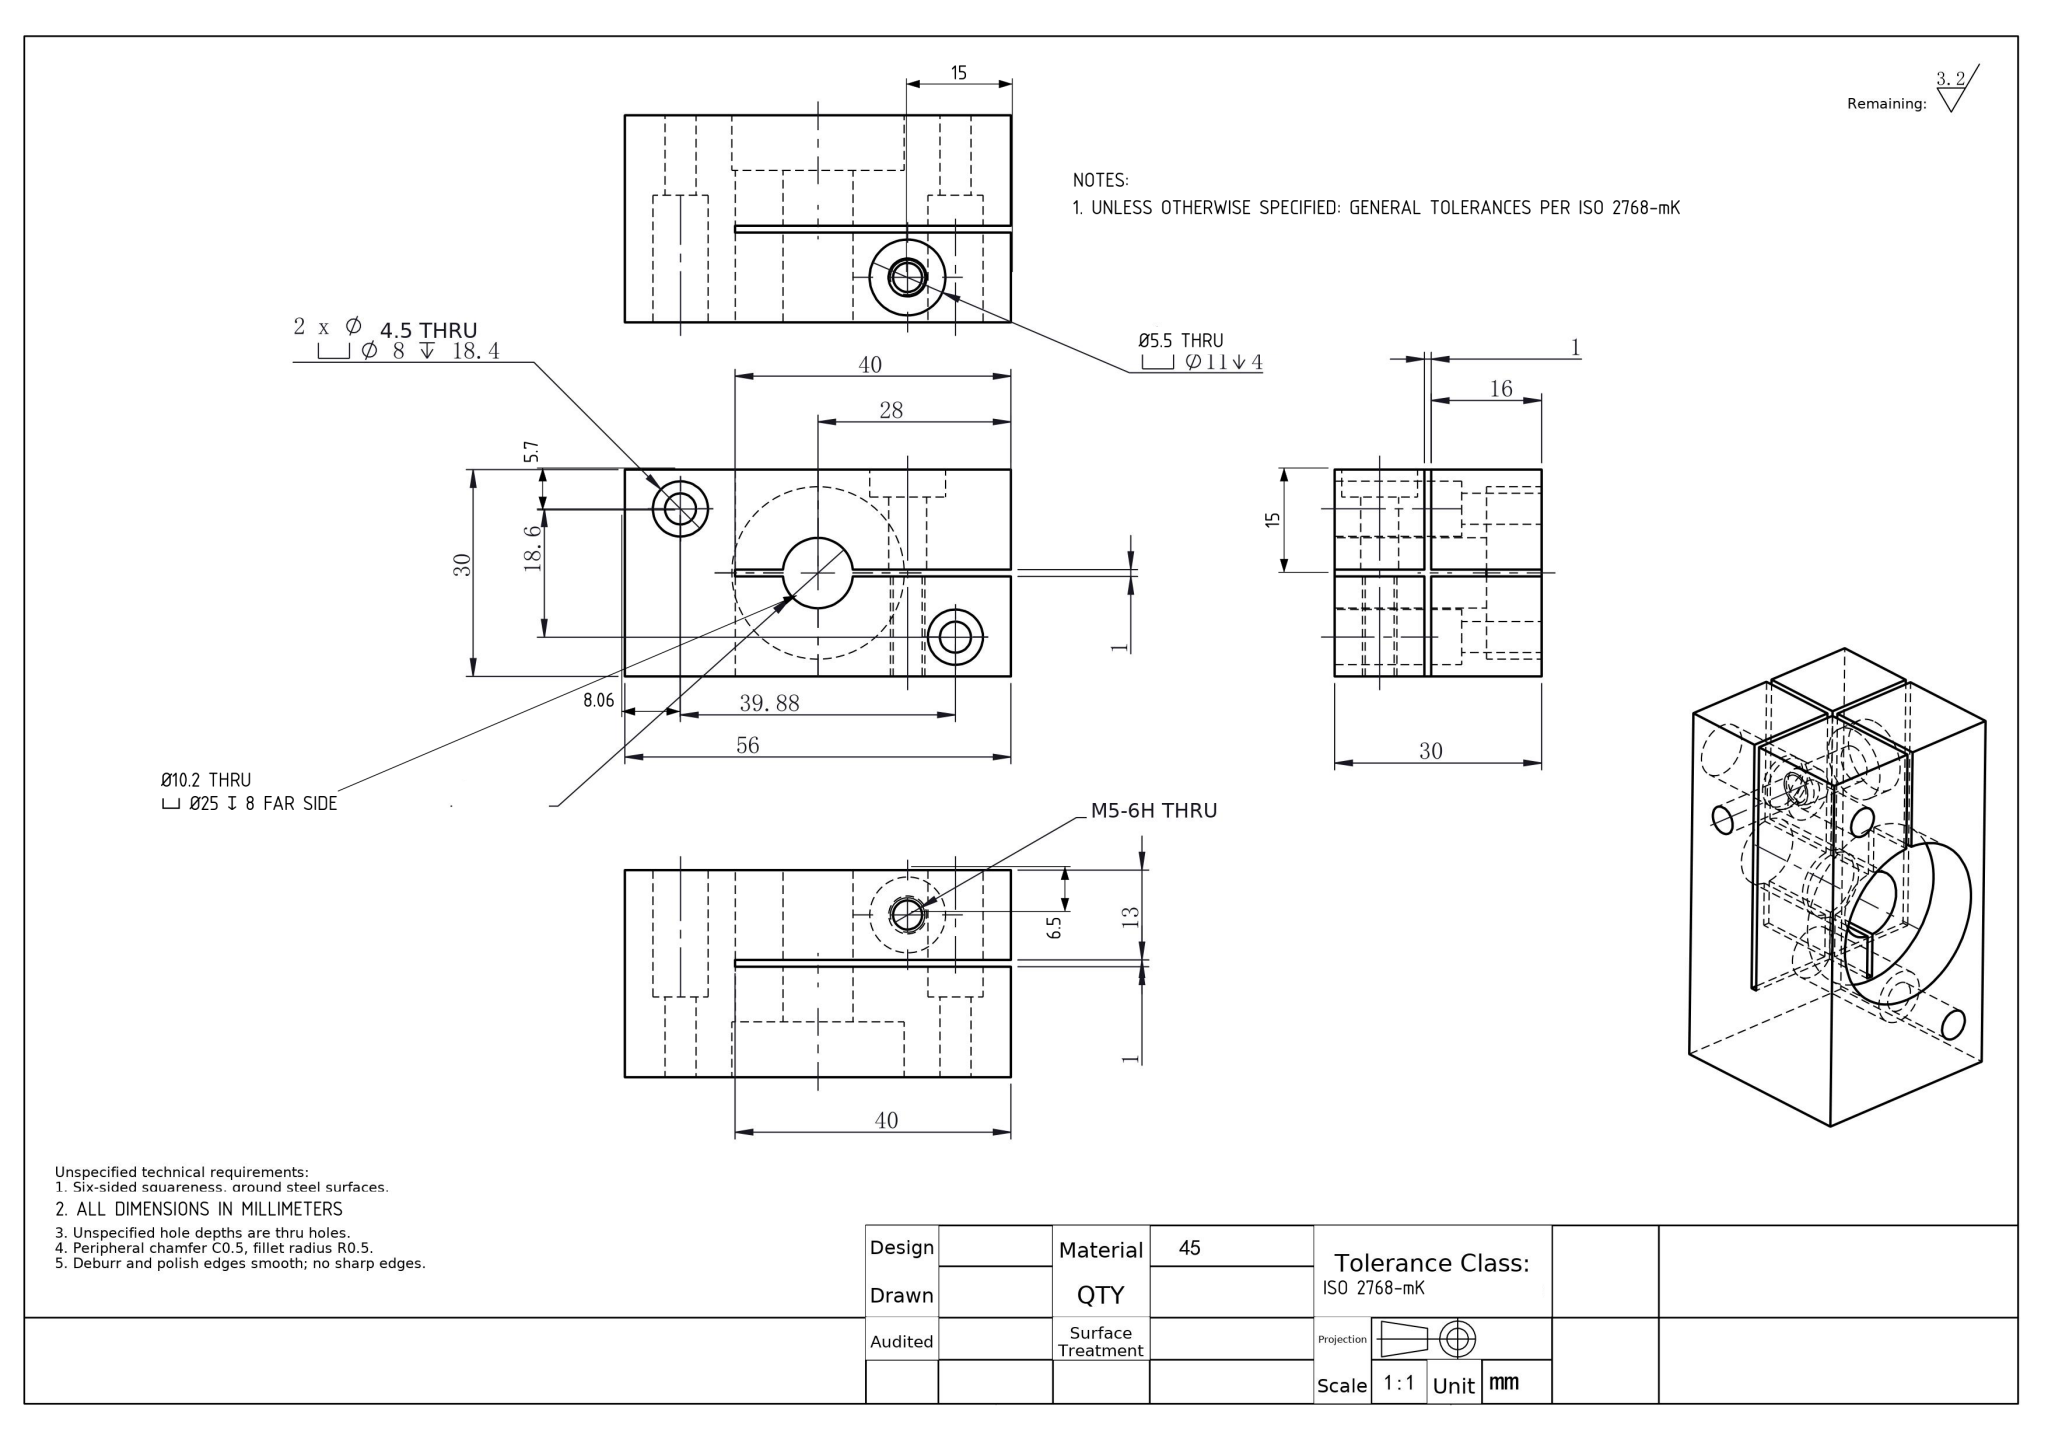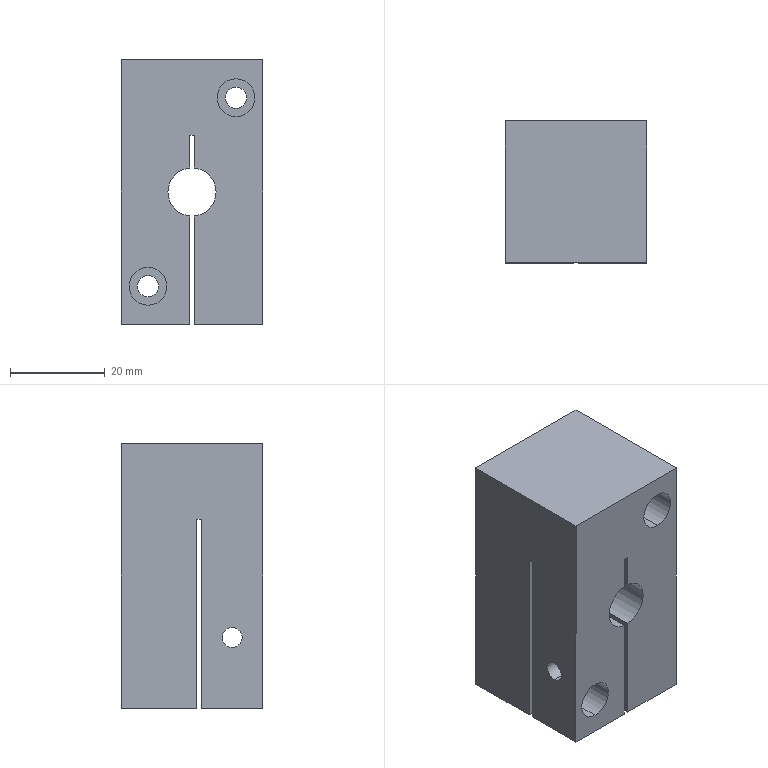Part | NX | mm | 1 solid | 48 faces | box 30 x 30 x 56 mm | volume 39808 mm3 | plane 26 | cylinder 22 | commonest cylinder face diameters 8 x6 4.5 x4 10.2 x4 4.2 x2 5.5 x2 11 x2 25 x2